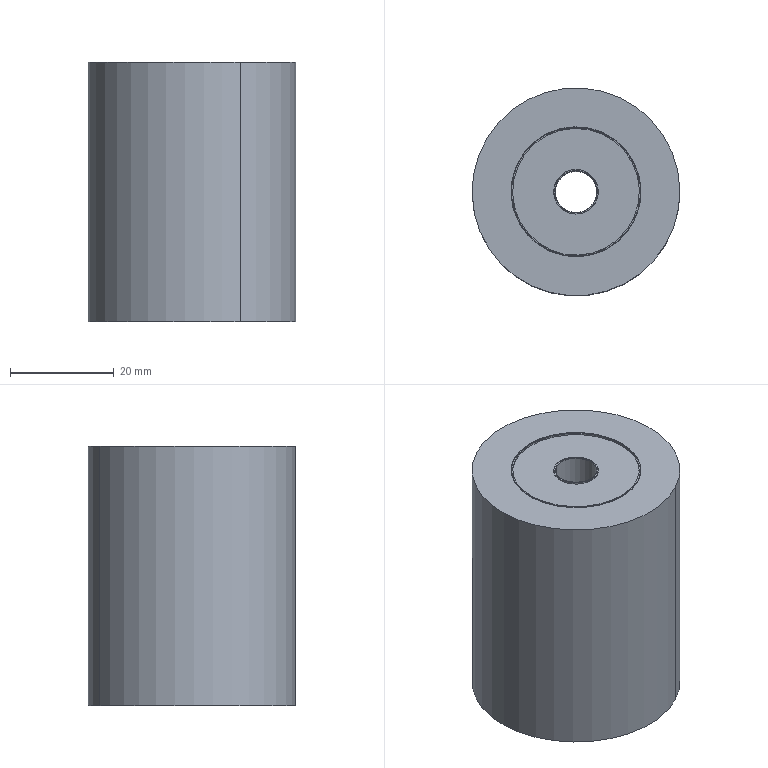Component | SolidWorks | 170423A4-ConveyorBeltIdlerAssembly1-1_170423A4-ENN02-D40-L50-1 | 1 solid | 58 faces | volume 48021 mm3 | cylinder 28 | spline 16 | plane 14 | commonest cylinder face diameters 8.6 x8 25 x4 24.4 x4 8 x4 21.4 x4 40 x2 22 x2